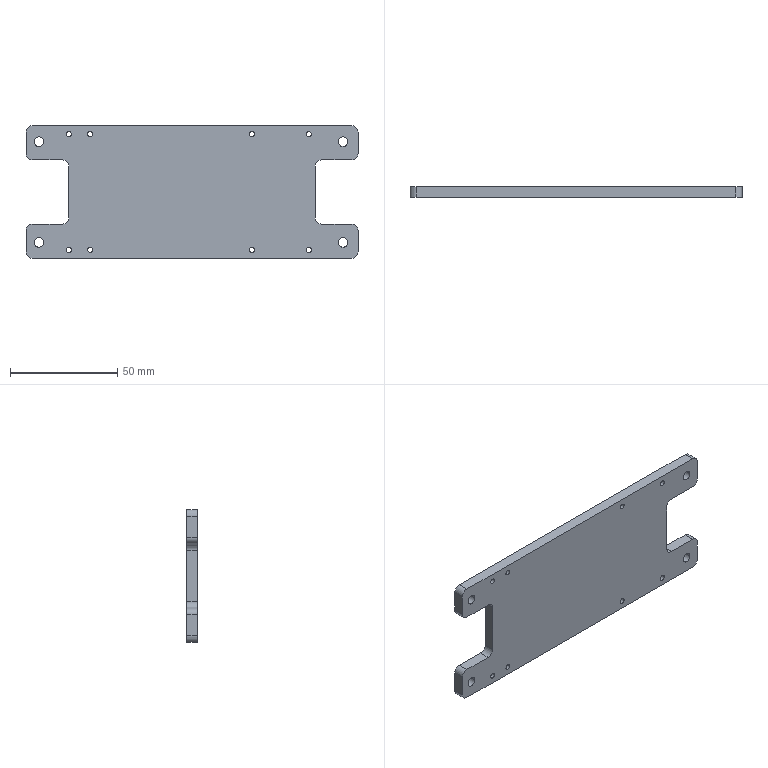CAM job | Mastercam | mm | 8 operations | part box 155 x 5 x 62
1. Facing | 24 - 100 平铣刀
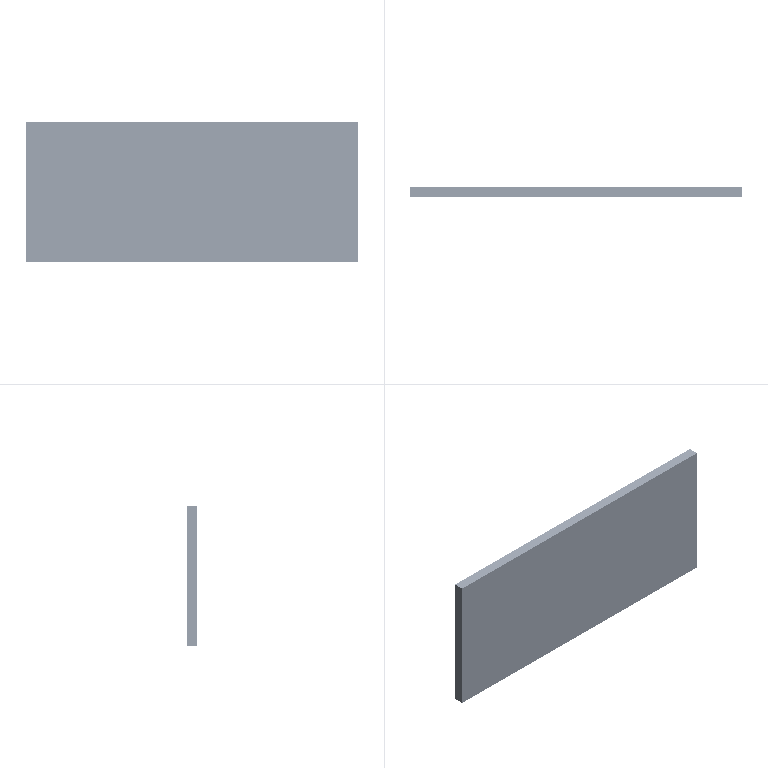2. 2D High Speed (2D Dynamic Mill) | 10 - 10 平铣刀
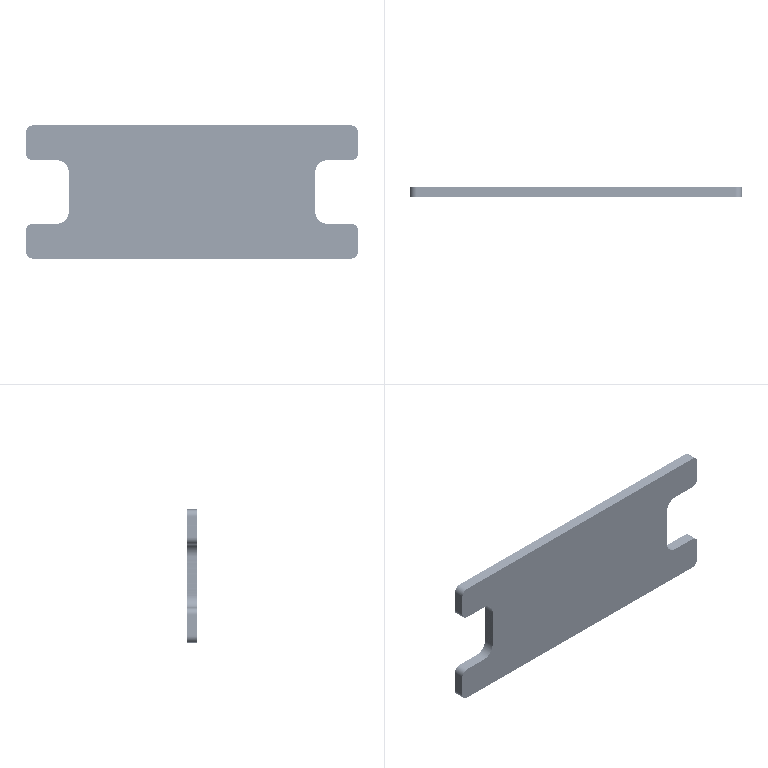3. Contour (Remachining) | 6 - 6 平铣刀
4. Contour (2D) | 6 - 6 平铣刀
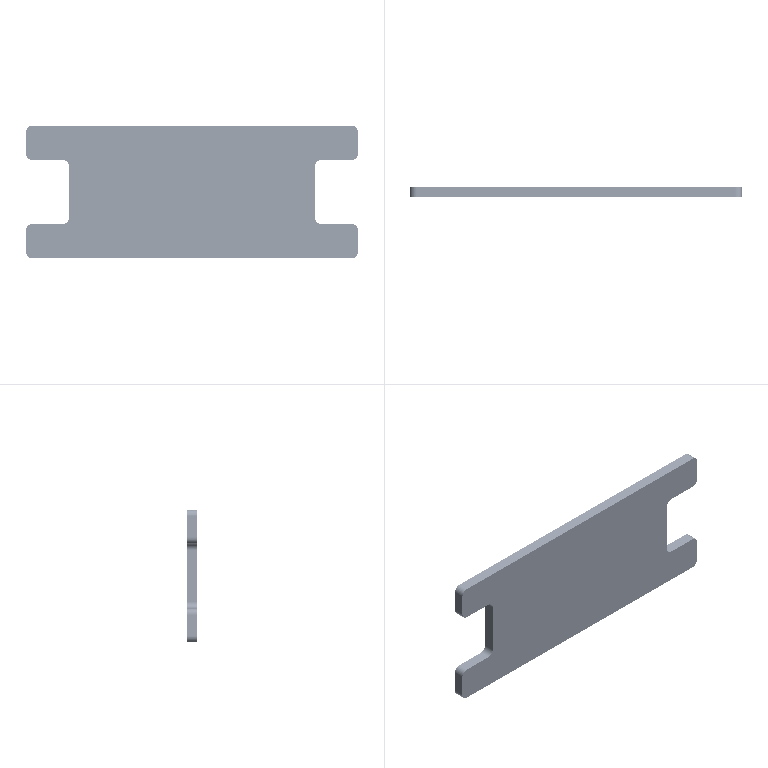5. Drill/Counterbore | 7 - 4 倒角刀
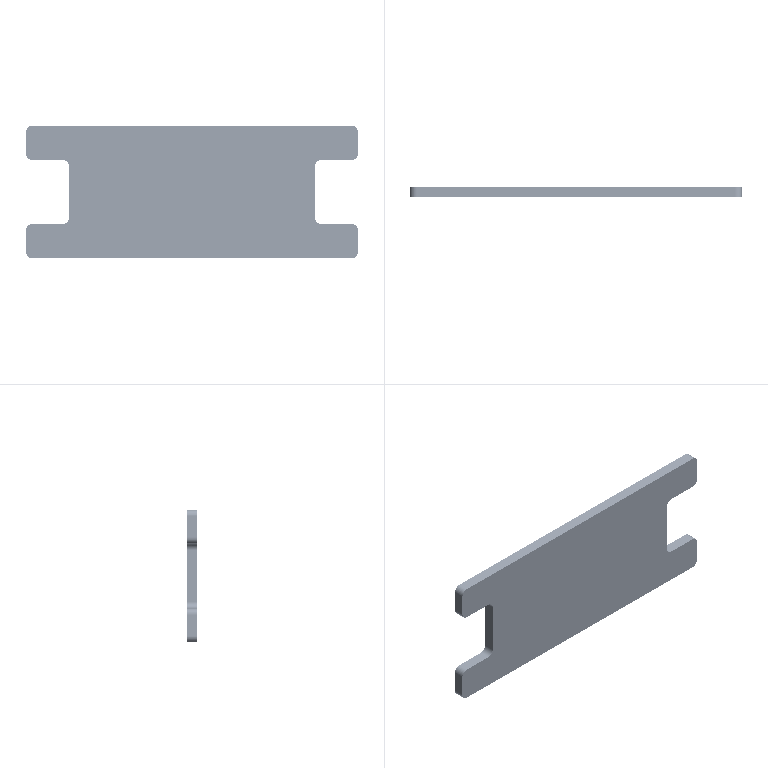6. Contour (2D chamfer) | 7 - 4 倒角刀
7. Facing | 24 - 100 平铣刀
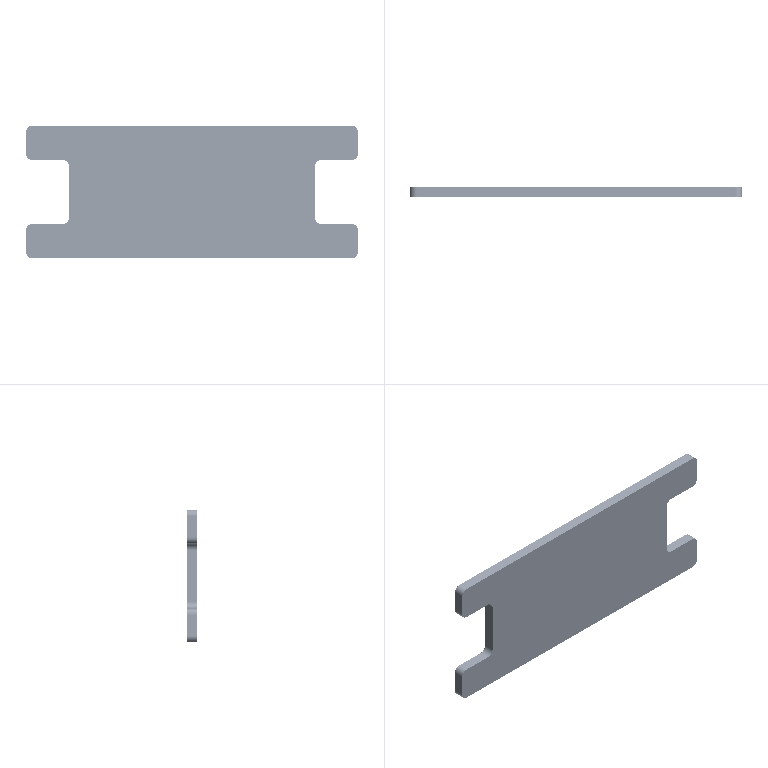8. Contour (2D chamfer) | 7 - 4 倒角刀